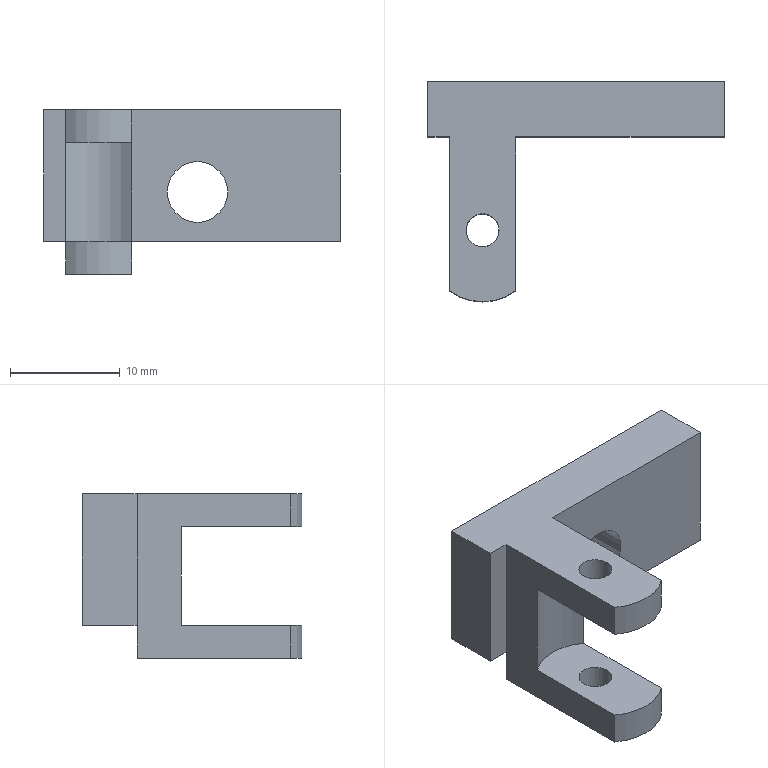Component | NX | 15_GAUGE_HOLDER | 1 solid | 19 faces | volume 2167 mm3 | plane 13 | cylinder 6 | commonest cylinder face diameters 10 x3 3 x2 5.5 x1